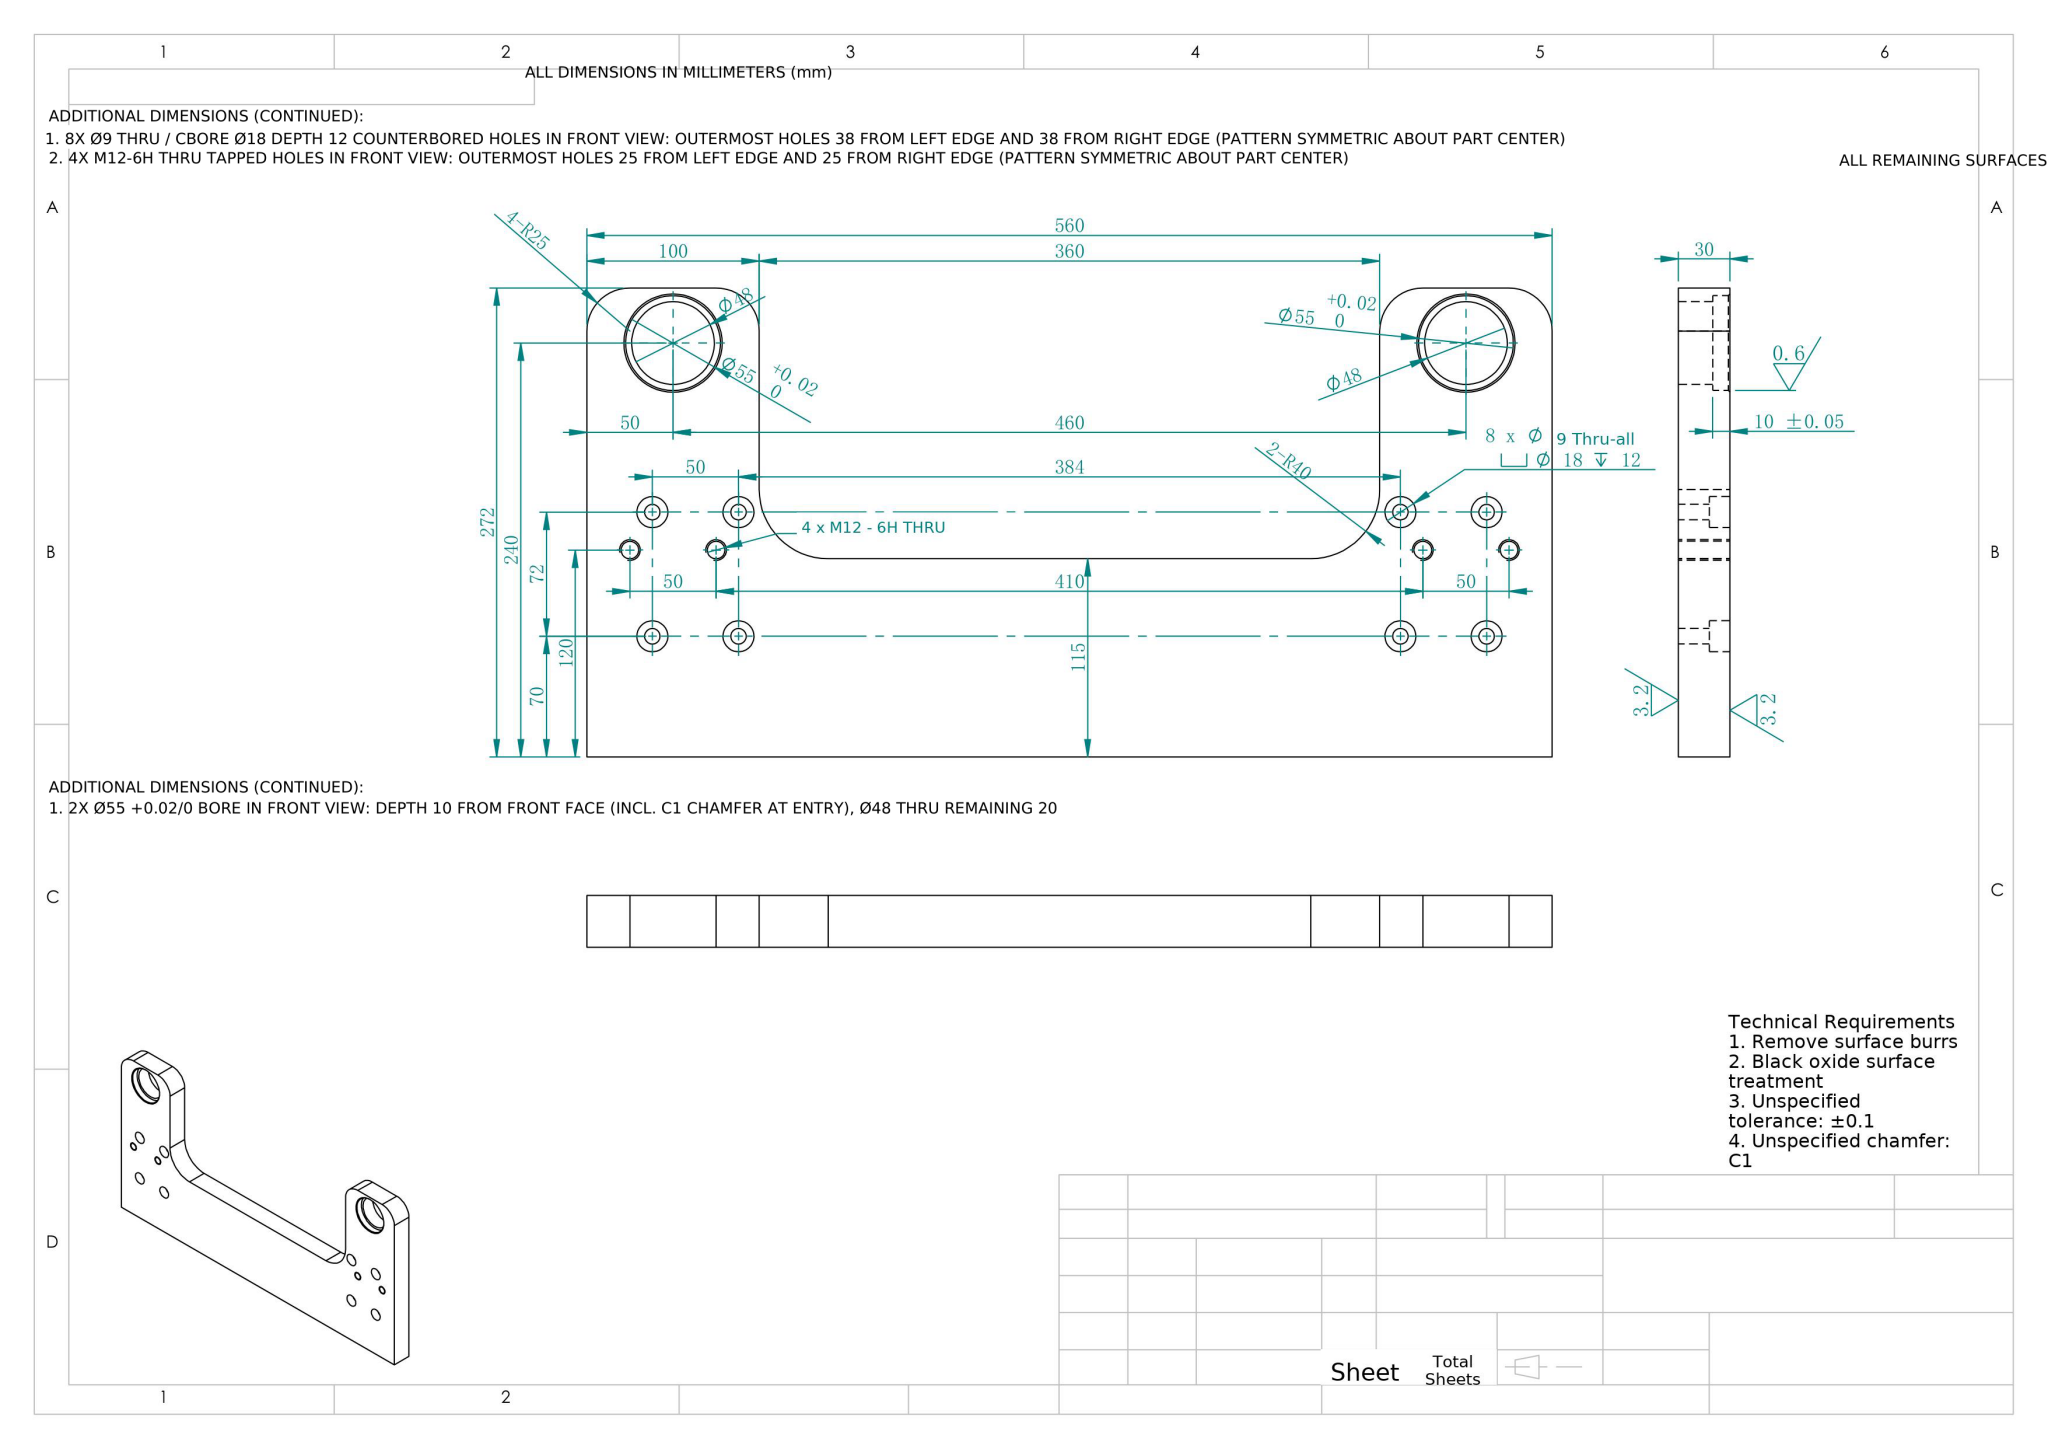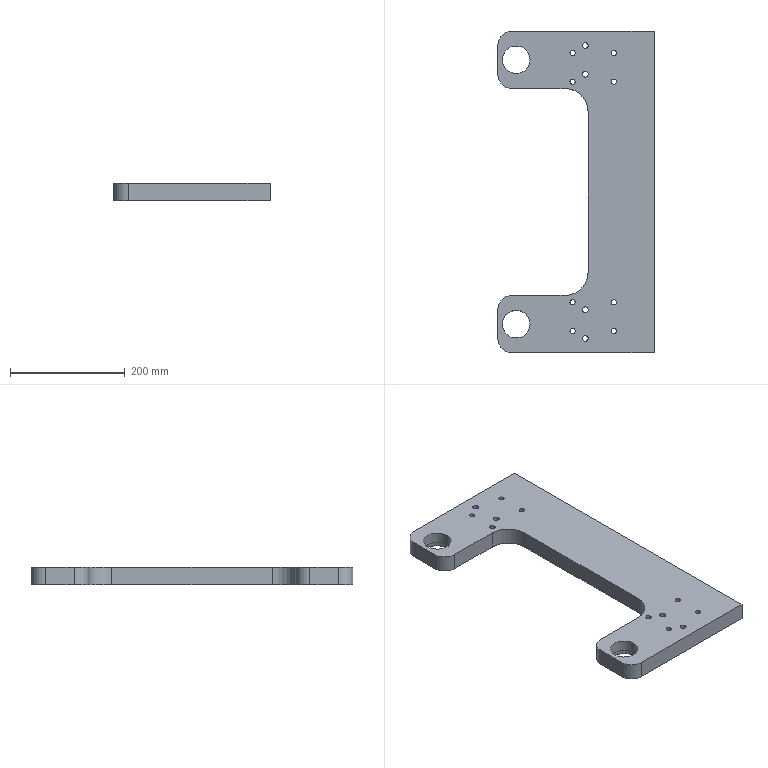Part | NX | mm | 1 solid | 78 faces | box 272 x 560 x 30 mm | volume 2715037 mm3 | cylinder 54 | plane 20 | cone 4 | commonest cylinder face diameters 18 x16 9 x16 10.2 x8 48 x4 55 x4 50 x4 80 x2